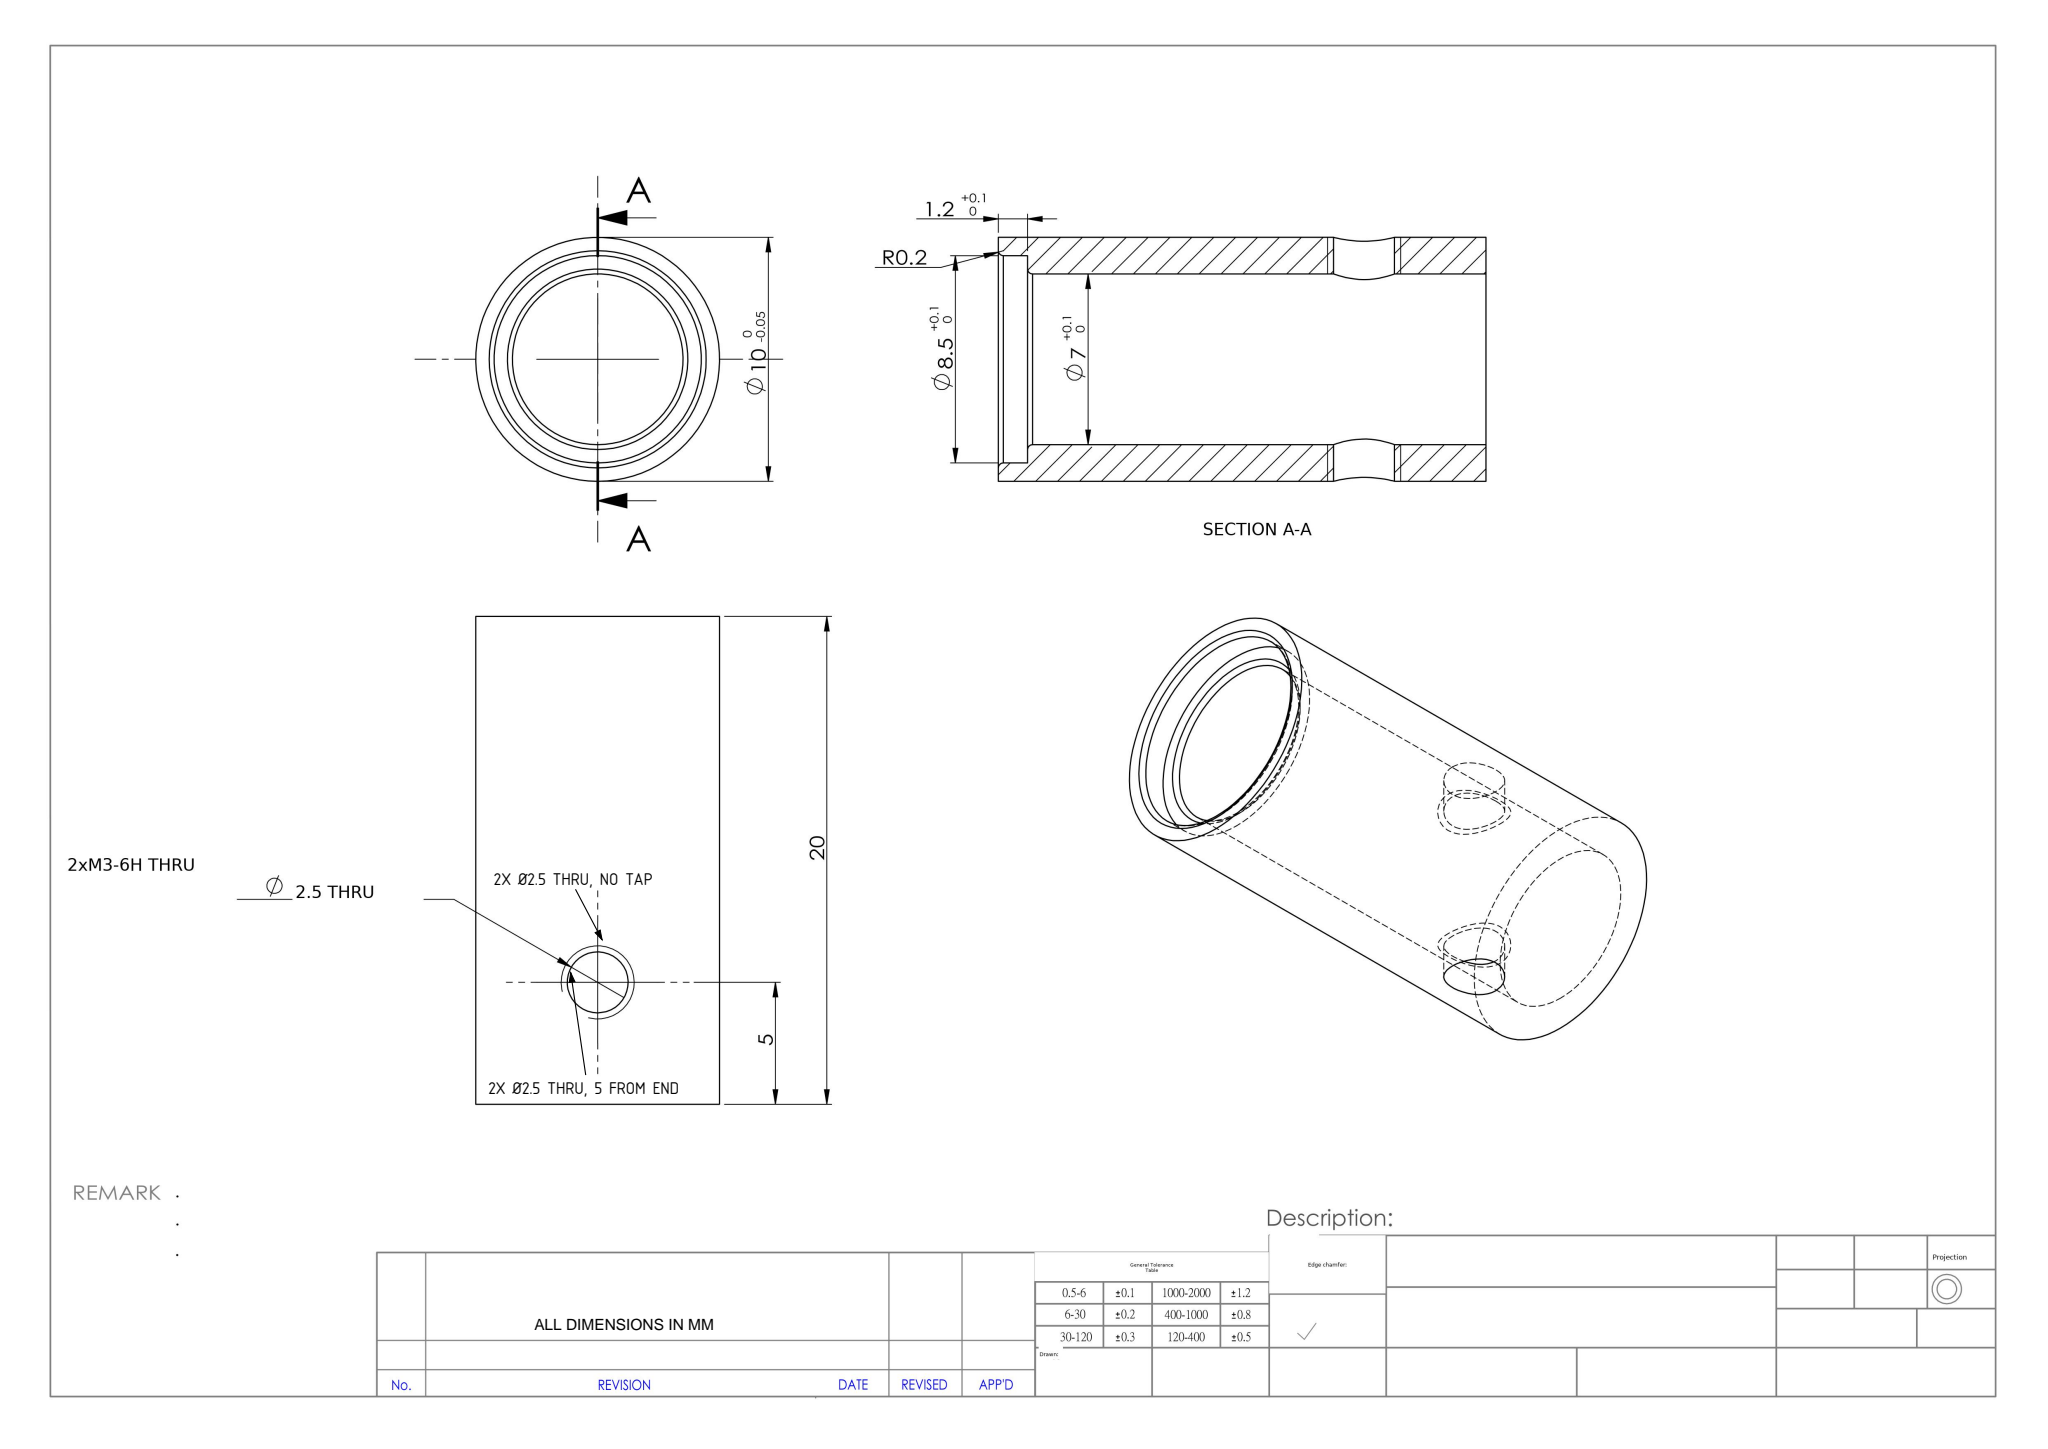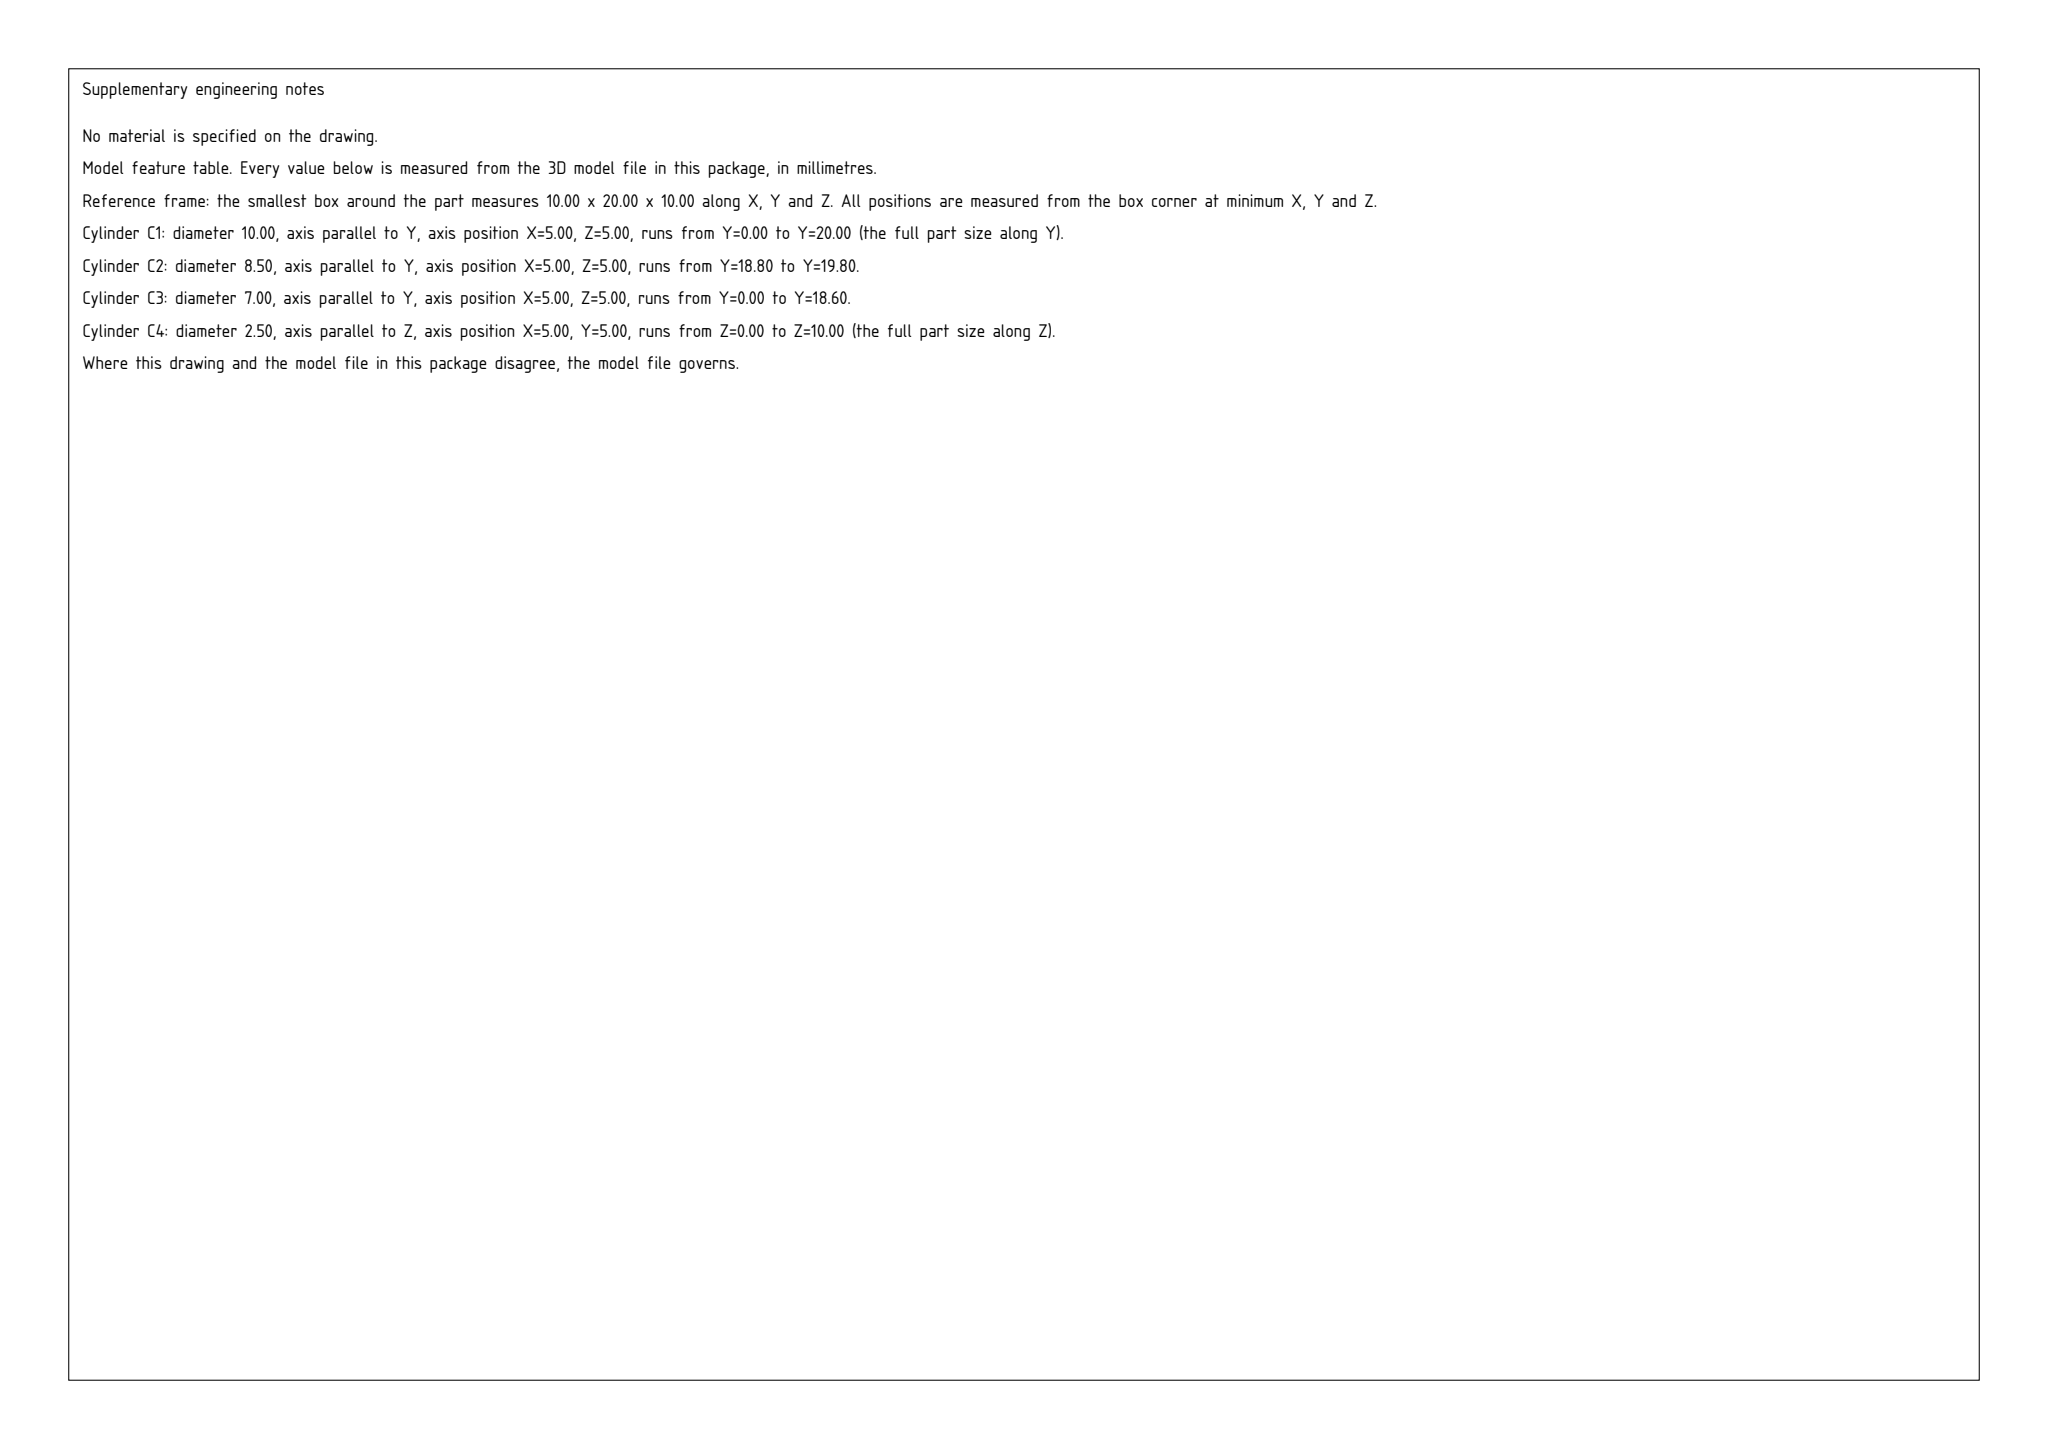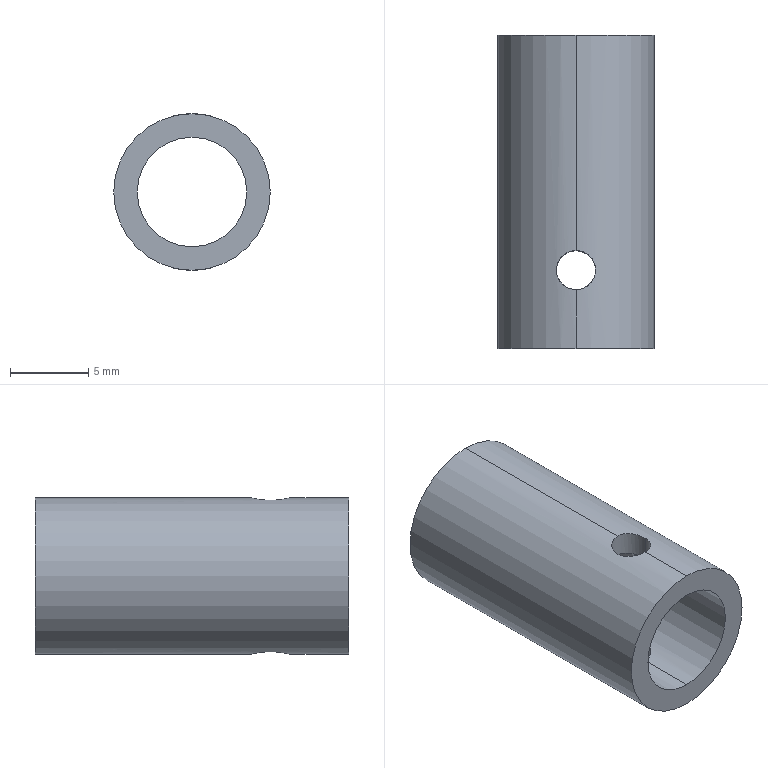Part | SolidWorks | mm | 1 solid | 17 faces | box 10 x 20 x 10 mm | volume 764 mm3 | cylinder 10 | torus 4 | plane 3 | commonest cylinder face diameters 2.5 x4 8.5 x2 10 x2 7 x2
Drawing notes:
2X Ø2.5 THRU WALL - NOT TAPPED (DELETE 2xM3-6H NOTE) | from the solid: Two Ø2.5 bores on z axis at x=5, y=5 (z 0-1.7 and 8.3-10); no thread/cone geometry in STEP
2X Ø2.5 THRU, ON C/L, 5 FROM BOTTOM END FACE | from the solid: Ø2.5 holes, axis z, located x=5.0 (Ø10 c/l), y=5.0 from y=0 end face; part length 20
build123d program:
from build123d import *

# Parameters (mm, degrees)
SKETCH7_R           = 5
BOSS_EXTRUDE3_DEPTH = 20
SKETCH8_R           = 3.5
CUT_EXTRUDE3_DEPTH  = 22.213
SKETCH9_R           = 4.25
CUT_EXTRUDE4_DEPTH  = 1.2
SKETCH14_W          = 1.25
SKETCH14_H          = 5
M3_TAPPED_HOLE2_D   = 2.5
FILLET1_R           = 0.2


with BuildPart() as part:
    # Sketch7 → Boss-Extrude3 (new body)
    with BuildSketch(Plane(origin=(0, 0, 0), x_dir=(1, 0, 0), z_dir=(0, 1, 0))):
        with Locations(Location((0, 0, 0), (0, 0, 270))):
            Circle(SKETCH7_R)
    extrude(amount=BOSS_EXTRUDE3_DEPTH)

    # Sketch8 → Cut-Extrude3 (cut, through all)
    with BuildSketch(Plane(origin=(0, 20, 0), x_dir=(1, 0, 0), z_dir=(0, 1, 0))):
        with Locations(Location((0, 0, 0), (0, 0, 270))):
            Circle(SKETCH8_R)
    extrude(amount=-CUT_EXTRUDE3_DEPTH, mode=Mode.SUBTRACT)

    # Sketch9 → Cut-Extrude4 (cut)
    with BuildSketch(Plane(origin=(0, 20, 0), x_dir=(1, 0, 0), z_dir=(0, 1, 0))):
        with Locations(Location((0, 0, 0), (0, 0, 270))):
            Circle(SKETCH9_R)
    extrude(amount=-CUT_EXTRUDE4_DEPTH, mode=Mode.SUBTRACT)

    # Sketch14 → M3 Tapped Hole1 (revolve, cut)
    with BuildSketch(Plane(origin=(0, 5, 0), x_dir=(0, 1, 0), z_dir=(1, 0, 0))):
        with Locations((0.625, 2.5)):
            Rectangle(SKETCH14_W, SKETCH14_H)
    revolve(axis=Axis((0, 5, -6.35), (0, 0, 1)), mode=Mode.SUBTRACT)

    # M3 Tapped Hole2 (through all)
    with Locations(Plane.XY):
        with Locations((0, 5)):
            Hole(M3_TAPPED_HOLE2_D / 2)

    # Fillet1
    fillet1_edges = [part.edges().sort_by_distance(p)[0] for p in [
        (0, 20, -4.25),
        (0, 18.8, -3.5),
    ]]
    fillet(fillet1_edges, radius=FILLET1_R)


solid = part.part
STEP:
#1=CARTESIAN_POINT('',(0.,18.8,-3.7));
#2=VERTEX_POINT('',#1);
#3=CARTESIAN_POINT('',(0.,18.8,3.7));
#4=VERTEX_POINT('',#3);
#5=CARTESIAN_POINT('',(0.,18.8,0.));
#6=DIRECTION('',(0.,-1.,0.));
#7=DIRECTION('',(0.,0.,1.));
#8=AXIS2_PLACEMENT_3D('',#5,#6,#7);
#9=CIRCLE('',#8,3.7);
#10=EDGE_CURVE('',#2,#4,#9,.T.);
#11=ORIENTED_EDGE('',*,*,#10,.F.);
#12=CARTESIAN_POINT('',(0.,18.6,-3.5));
#13=VERTEX_POINT('',#12);
#14=CARTESIAN_POINT('',(0.,18.6,-3.7));
#15=DIRECTION('',(1.,0.,0.));
#16=DIRECTION('',(0.,0.,-1.));
#17=AXIS2_PLACEMENT_3D('',#14,#15,#16);
#18=CIRCLE('',#17,0.2);
#19=EDGE_CURVE('',#2,#13,#18,.T.);
#20=ORIENTED_EDGE('',*,*,#19,.T.);
#21=CARTESIAN_POINT('',(0.,18.6,3.5));
#22=VERTEX_POINT('',#21);
#23=CARTESIAN_POINT('',(0.,18.6,0.));
#24=DIRECTION('',(0.,1.,0.));
#25=DIRECTION('',(0.,0.,1.));
#26=AXIS2_PLACEMENT_3D('',#23,#24,#25);
#27=CIRCLE('',#26,3.5);
#28=EDGE_CURVE('',#22,#13,#27,.T.);
#29=ORIENTED_EDGE('',*,*,#28,.F.);
#30=CARTESIAN_POINT('',(0.,18.6,3.7));
#31=DIRECTION('',(-1.,0.,0.));
#32=DIRECTION('',(0.,0.,1.));
#33=AXIS2_PLACEMENT_3D('',#30,#31,#32);
#34=CIRCLE('',#33,0.2);
#35=EDGE_CURVE('',#4,#22,#34,.T.);
#36=ORIENTED_EDGE('',*,*,#35,.F.);
#37=EDGE_LOOP('',(#11,#20,#29,#36));
#38=FACE_OUTER_BOUND('',#37,.T.);
#39=CARTESIAN_POINT('',(0.,18.6,0.));
#40=DIRECTION('',(0.,1.,0.));
#41=DIRECTION('',(0.,0.,1.));
#42=AXIS2_PLACEMENT_3D('',#39,#40,#41);
#43=TOROIDAL_SURFACE('',#42,3.7,0.2);
#44=ADVANCED_FACE('',(#38),#43,.T.);
#45=CARTESIAN_POINT('',(0.,20.,-4.45));
#46=VERTEX_POINT('',#45);
#47=CARTESIAN_POINT('',(0.,20.,4.45));
#48=VERTEX_POINT('',#47);
#49=CARTESIAN_POINT('',(0.,20.,0.));
#50=DIRECTION('',(0.,-1.,0.));
#51=DIRECTION('',(0.,0.,1.));
#52=AXIS2_PLACEMENT_3D('',#49,#50,#51);
#53=CIRCLE('',#52,4.45);
#54=EDGE_CURVE('',#46,#48,#53,.T.);
#55=ORIENTED_EDGE('',*,*,#54,.F.);
#56=CARTESIAN_POINT('',(0.,19.8,-4.25));
#57=VERTEX_POINT('',#56);
#58=CARTESIAN_POINT('',(0.,19.8,-4.45));
#59=DIRECTION('',(1.,0.,0.));
#60=DIRECTION('',(0.,0.,-1.));
#61=AXIS2_PLACEMENT_3D('',#58,#59,#60);
#62=CIRCLE('',#61,0.2);
#63=EDGE_CURVE('',#46,#57,#62,.T.);
#64=ORIENTED_EDGE('',*,*,#63,.T.);
#65=CARTESIAN_POINT('',(0.,19.8,4.25));
#66=VERTEX_POINT('',#65);
#67=CARTESIAN_POINT('',(0.,19.8,0.));
#68=DIRECTION('',(0.,1.,0.));
#69=DIRECTION('',(0.,0.,1.));
#70=AXIS2_PLACEMENT_3D('',#67,#68,#69);
#71=CIRCLE('',#70,4.25);
#72=EDGE_CURVE('',#66,#57,#71,.T.);
#73=ORIENTED_EDGE('',*,*,#72,.F.);
#74=CARTESIAN_POINT('',(0.,19.8,4.45));
#75=DIRECTION('',(-1.,0.,0.));
#76=DIRECTION('',(0.,0.,1.));
#77=AXIS2_PLACEMENT_3D('',#74,#75,#76);
#78=CIRCLE('',#77,0.2);
#79=EDGE_CURVE('',#48,#66,#78,.T.);
#80=ORIENTED_EDGE('',*,*,#79,.F.);
#81=EDGE_LOOP('',(#55,#64,#73,#80));
#82=FACE_OUTER_BOUND('',#81,.T.);
#83=CARTESIAN_POINT('',(0.,19.8,0.));
#84=DIRECTION('',(0.,1.,0.));
#85=DIRECTION('',(0.,0.,1.));
#86=AXIS2_PLACEMENT_3D('',#83,#84,#85);
#87=TOROIDAL_SURFACE('',#86,4.45,0.2);
#88=ADVANCED_FACE('',(#82),#87,.T.);
#89=CARTESIAN_POINT('',(-1.25,5.,-4.841));
#90=VERTEX_POINT('',#89);
#91=CARTESIAN_POINT('',(0.,3.75,-5.));
#92=VERTEX_POINT('',#91);
#93=CARTESIAN_POINT('',(-1.25,5.,-4.841));
#94=CARTESIAN_POINT('',(-1.25,4.918,-4.841));
#95=CARTESIAN_POINT('',(-1.242,4.835,-4.843));
#96=CARTESIAN_POINT('',(-1.21,4.674,-4.852));
#97=CARTESIAN_POINT('',(-1.186,4.596,-4.857));
#98=CARTESIAN_POINT('',(-1.091,4.369,-4.88));
#99=CARTESIAN_POINT('',(-0.9993,4.231,-4.901));
#100=CARTESIAN_POINT('',(-0.8256,4.058,-4.932));
#101=CARTESIAN_POINT('',(-0.7628,4.006,-4.942));
#102=CARTESIAN_POINT('',(-0.6277,3.916,-4.961));
#103=CARTESIAN_POINT('',(-0.5545,3.877,-4.97));
#104=CARTESIAN_POINT('',(-0.3282,3.783,-4.992));
#105=CARTESIAN_POINT('',(-0.1635,3.75,-5.));
#106=CARTESIAN_POINT('',(0.,3.75,-5.));
#107=B_SPLINE_CURVE_WITH_KNOTS('',3,(#93,#94,#95,#96,#97,#98,#99,#100,#101,#102,#103,#104,#105,#106),.UNSPECIFIED.,.F.,.F.,(4,2,2,2,2,2,4),(0.001962,0.002208,0.002453,0.002943,0.003188,0.003433,0.003924),.UNSPECIFIED.);
#108=EDGE_CURVE('',#90,#92,#107,.T.);
#109=ORIENTED_EDGE('',*,*,#108,.F.);
#110=CARTESIAN_POINT('',(-1.25,5.,-3.269));
#111=VERTEX_POINT('',#110);
#112=CARTESIAN_POINT('',(-1.25,5.,0.));
#113=DIRECTION('',(0.,0.,1.));
#114=VECTOR('',#113,1000.);
#115=LINE('',#112,#114);
#116=EDGE_CURVE('',#90,#111,#115,.T.);
#117=ORIENTED_EDGE('',*,*,#116,.T.);
#118=CARTESIAN_POINT('',(-0.,3.75,-3.5));
#119=VERTEX_POINT('',#118);
#120=CARTESIAN_POINT('',(-0.,3.75,-3.5));
#121=CARTESIAN_POINT('',(-0.08231,3.75,-3.5));
#122=CARTESIAN_POINT('',(-0.1659,3.758,-3.497));
#123=CARTESIAN_POINT('',(-0.3268,3.791,-3.486));
#124=CARTESIAN_POINT('',(-0.405,3.815,-3.477));
#125=CARTESIAN_POINT('',(-0.6334,3.91,-3.446));
#126=CARTESIAN_POINT('',(-0.7701,4.002,-3.416));
#127=CARTESIAN_POINT('',(-0.9421,4.174,-3.371));
#128=CARTESIAN_POINT('',(-0.9934,4.237,-3.356));
#129=CARTESIAN_POINT('',(-1.084,4.372,-3.328));
#130=CARTESIAN_POINT('',(-1.123,4.445,-3.315));
#131=CARTESIAN_POINT('',(-1.217,4.67,-3.282));
#132=CARTESIAN_POINT('',(-1.25,4.836,-3.269));
#133=CARTESIAN_POINT('',(-1.25,5.,-3.269));
#134=B_SPLINE_CURVE_WITH_KNOTS('',3,(#120,#121,#122,#123,#124,#125,#126,#127,#128,#129,#130,#131,#132,#133),.UNSPECIFIED.,.F.,.F.,(4,2,2,2,2,2,4),(0.001971,0.002217,0.002463,0.002956,0.003202,0.003448,0.003941),.UNSPECIFIED.);
#135=EDGE_CURVE('',#119,#111,#134,.T.);
#136=ORIENTED_EDGE('',*,*,#135,.F.);
#137=CARTESIAN_POINT('',(1.25,5.,-3.269));
#138=VERTEX_POINT('',#137);
#139=CARTESIAN_POINT('',(1.25,5.,-3.269));
#140=CARTESIAN_POINT('',(1.25,4.833,-3.269));
#141=CARTESIAN_POINT('',(1.217,4.67,-3.282));
#142=CARTESIAN_POINT('',(1.091,4.368,-3.326));
#143=CARTESIAN_POINT('',(0.9979,4.23,-3.357));
#144=CARTESIAN_POINT('',(0.7692,4.002,-3.416));
#145=CARTESIAN_POINT('',(0.6308,3.909,-3.446));
#146=CARTESIAN_POINT('',(0.3302,3.783,-3.488));
#147=CARTESIAN_POINT('',(0.1647,3.75,-3.5));
#148=CARTESIAN_POINT('',(-0.,3.75,-3.5));
#149=B_SPLINE_CURVE_WITH_KNOTS('',3,(#139,#140,#141,#142,#143,#144,#145,#146,#147,#148),.UNSPECIFIED.,.F.,.F.,(4,2,2,2,4),(0.,0.0004927,0.0009855,0.001478,0.001971),.UNSPECIFIED.);
#150=EDGE_CURVE('',#138,#119,#149,.T.);
#151=ORIENTED_EDGE('',*,*,#150,.F.);
#152=CARTESIAN_POINT('',(1.25,5.,-4.841));
#153=VERTEX_POINT('',#152);
#154=CARTESIAN_POINT('',(1.25,5.,0.));
#155=DIRECTION('',(0.,0.,1.));
#156=VECTOR('',#155,1000.);
#157=LINE('',#154,#156);
#158=EDGE_CURVE('',#153,#138,#157,.T.);
#159=ORIENTED_EDGE('',*,*,#158,.F.);
#160=CARTESIAN_POINT('',(0.,3.75,-5.));
#161=CARTESIAN_POINT('',(0.1635,3.75,-5.));
#162=CARTESIAN_POINT('',(0.3287,3.783,-4.991));
#163=CARTESIAN_POINT('',(0.6298,3.908,-4.962));
#164=CARTESIAN_POINT('',(0.7684,4.001,-4.942));
#165=CARTESIAN_POINT('',(0.999,4.231,-4.901));
#166=CARTESIAN_POINT('',(1.091,4.368,-4.88));
#167=CARTESIAN_POINT('',(1.217,4.672,-4.85));
#168=CARTESIAN_POINT('',(1.25,4.835,-4.841));
#169=CARTESIAN_POINT('',(1.25,5.,-4.841));
#170=B_SPLINE_CURVE_WITH_KNOTS('',3,(#160,#161,#162,#163,#164,#165,#166,#167,#168,#169),.UNSPECIFIED.,.F.,.F.,(4,2,2,2,4),(0.003924,0.004414,0.004905,0.005395,0.005885),.UNSPECIFIED.);
#171=EDGE_CURVE('',#92,#153,#170,.T.);
#172=ORIENTED_EDGE('',*,*,#171,.F.);
#173=EDGE_LOOP('',(#109,#117,#136,#151,#159,#172));
#174=FACE_OUTER_BOUND('',#173,.T.);
#175=CARTESIAN_POINT('',(0.,5.,0.));
#176=DIRECTION('',(0.,0.,1.));
#177=DIRECTION('',(1.,0.,0.));
#178=AXIS2_PLACEMENT_3D('',#175,#176,#177);
#179=CYLINDRICAL_SURFACE('',#178,1.25);
#180=ADVANCED_FACE('',(#174),#179,.F.);
#181=CARTESIAN_POINT('',(1.25,5.,4.841));
#182=VERTEX_POINT('',#181);
#183=CARTESIAN_POINT('',(0.,3.75,5.));
#184=VERTEX_POINT('',#183);
#185=CARTESIAN_POINT('',(1.25,5.,4.841));
#186=CARTESIAN_POINT('',(1.25,4.918,4.841));
#187=CARTESIAN_POINT('',(1.242,4.836,4.843));
#188=CARTESIAN_POINT('',(1.21,4.676,4.851));
#189=CARTESIAN_POINT('',(1.186,4.596,4.857));
#190=CARTESIAN_POINT('',(1.092,4.37,4.88));
#191=CARTESIAN_POINT('',(0.9989,4.231,4.901));
#192=CARTESIAN_POINT('',(0.7696,4.002,4.942));
#193=CARTESIAN_POINT('',(0.6309,3.909,4.962));
#194=CARTESIAN_POINT('',(0.3301,3.783,4.991));
#195=CARTESIAN_POINT('',(0.1658,3.75,5.));
#196=CARTESIAN_POINT('',(0.,3.75,5.));
#197=B_SPLINE_CURVE_WITH_KNOTS('',3,(#185,#186,#187,#188,#189,#190,#191,#192,#193,#194,#195,#196),.UNSPECIFIED.,.F.,.F.,(4,2,2,2,2,4),(0.005885,0.006131,0.006376,0.006866,0.007356,0.007846),.UNSPECIFIED.);
#198=EDGE_CURVE('',#182,#184,#197,.T.);
#199=ORIENTED_EDGE('',*,*,#198,.F.);
#200=CARTESIAN_POINT('',(1.25,5.,3.269));
#201=VERTEX_POINT('',#200);
#202=CARTESIAN_POINT('',(1.25,5.,0.));
#203=DIRECTION('',(0.,0.,-1.));
#204=VECTOR('',#203,1000.);
#205=LINE('',#202,#204);
#206=EDGE_CURVE('',#182,#201,#205,.T.);
#207=ORIENTED_EDGE('',*,*,#206,.T.);
#208=CARTESIAN_POINT('',(0.,3.75,3.5));
#209=VERTEX_POINT('',#208);
#210=CARTESIAN_POINT('',(0.,3.75,3.5));
#211=CARTESIAN_POINT('',(0.1667,3.75,3.5));
#212=CARTESIAN_POINT('',(0.3302,3.783,3.488));
#213=CARTESIAN_POINT('',(0.6325,3.909,3.446));
#214=CARTESIAN_POINT('',(0.7703,4.002,3.416));
#215=CARTESIAN_POINT('',(0.9988,4.231,3.357));
#216=CARTESIAN_POINT('',(1.092,4.37,3.326));
#217=CARTESIAN_POINT('',(1.217,4.67,3.282));
#218=CARTESIAN_POINT('',(1.25,4.835,3.269));
#219=CARTESIAN_POINT('',(1.25,5.,3.269));
#220=B_SPLINE_CURVE_WITH_KNOTS('',3,(#210,#211,#212,#213,#214,#215,#216,#217,#218,#219),.UNSPECIFIED.,.F.,.F.,(4,2,2,2,4),(0.,0.0004928,0.0009856,0.001478,0.001971),.UNSPECIFIED.);
#221=EDGE_CURVE('',#209,#201,#220,.T.);
#222=ORIENTED_EDGE('',*,*,#221,.F.);
#223=CARTESIAN_POINT('',(-1.25,5.,3.269));
#224=VERTEX_POINT('',#223);
#225=CARTESIAN_POINT('',(-1.25,5.,3.269));
#226=CARTESIAN_POINT('',(-1.25,4.835,3.269));
#227=CARTESIAN_POINT('',(-1.217,4.67,3.282));
#228=CARTESIAN_POINT('',(-1.091,4.369,3.326));
#229=CARTESIAN_POINT('',(-0.9986,4.231,3.357));
#230=CARTESIAN_POINT('',(-0.7693,4.002,3.416));
#231=CARTESIAN_POINT('',(-0.6323,3.909,3.446));
#232=CARTESIAN_POINT('',(-0.3293,3.783,3.488));
#233=CARTESIAN_POINT('',(-0.1667,3.75,3.5));
#234=CARTESIAN_POINT('',(0.,3.75,3.5));
#235=B_SPLINE_CURVE_WITH_KNOTS('',3,(#225,#226,#227,#228,#229,#230,#231,#232,#233,#234),.UNSPECIFIED.,.F.,.F.,(4,2,2,2,4),(0.005911,0.006403,0.006896,0.007388,0.007881),.UNSPECIFIED.);
#236=EDGE_CURVE('',#224,#209,#235,.T.);
#237=ORIENTED_EDGE('',*,*,#236,.F.);
#238=CARTESIAN_POINT('',(-1.25,5.,4.841));
#239=VERTEX_POINT('',#238);
#240=CARTESIAN_POINT('',(-1.25,5.,0.));
#241=DIRECTION('',(0.,0.,-1.));
#242=VECTOR('',#241,1000.);
#243=LINE('',#240,#242);
#244=EDGE_CURVE('',#239,#224,#243,.T.);
#245=ORIENTED_EDGE('',*,*,#244,.F.);
#246=CARTESIAN_POINT('',(0.,3.75,5.));
#247=CARTESIAN_POINT('',(-0.1659,3.75,5.));
#248=CARTESIAN_POINT('',(-0.3287,3.783,4.991));
#249=CARTESIAN_POINT('',(-0.6313,3.909,4.962));
#250=CARTESIAN_POINT('',(-0.7695,4.002,4.942));
#251=CARTESIAN_POINT('',(-0.9991,4.231,4.901));
#252=CARTESIAN_POINT('',(-1.092,4.37,4.88));
#253=CARTESIAN_POINT('',(-1.217,4.671,4.85));
#254=CARTESIAN_POINT('',(-1.25,4.836,4.841));
#255=CARTESIAN_POINT('',(-1.25,5.,4.841));
#256=B_SPLINE_CURVE_WITH_KNOTS('',3,(#246,#247,#248,#249,#250,#251,#252,#253,#254,#255),.UNSPECIFIED.,.F.,.F.,(4,2,2,2,4),(0.,0.0004906,0.0009812,0.001472,0.001962),.UNSPECIFIED.);
#257=EDGE_CURVE('',#184,#239,#256,.T.);
#258=ORIENTED_EDGE('',*,*,#257,.F.);
#259=EDGE_LOOP('',(#199,#207,#222,#237,#245,#258));
#260=FACE_OUTER_BOUND('',#259,.T.);
#261=CARTESIAN_POINT('',(0.,5.,0.));
#262=DIRECTION('',(0.,0.,-1.));
#263=DIRECTION('',(-1.,0.,0.));
#264=AXIS2_PLACEMENT_3D('',#261,#262,#263);
#265=CYLINDRICAL_SURFACE('',#264,1.25);
#266=ADVANCED_FACE('',(#260),#265,.F.);
#267=CARTESIAN_POINT('',(0.,18.8,-4.25));
#268=VERTEX_POINT('',#267);
#269=CARTESIAN_POINT('',(0.,18.8,4.25));
#270=VERTEX_POINT('',#269);
#271=CARTESIAN_POINT('',(0.,18.8,0.));
#272=DIRECTION('',(0.,1.,0.));
#273=DIRECTION('',(0.,0.,1.));
#274=AXIS2_PLACEMENT_3D('',#271,#272,#273);
#275=CIRCLE('',#274,4.25);
#276=EDGE_CURVE('',#268,#270,#275,.T.);
#277=ORIENTED_EDGE('',*,*,#276,.F.);
#278=CARTESIAN_POINT('',(0.,18.8,-4.25));
#279=DIRECTION('',(0.,1.,0.));
#280=VECTOR('',#279,1000.);
#281=LINE('',#278,#280);
#282=EDGE_CURVE('',#268,#57,#281,.T.);
#283=ORIENTED_EDGE('',*,*,#282,.T.);
#284=CARTESIAN_POINT('',(0.,19.8,0.));
#285=DIRECTION('',(0.,1.,0.));
#286=DIRECTION('',(0.,0.,1.));
#287=AXIS2_PLACEMENT_3D('',#284,#285,#286);
#288=CIRCLE('',#287,4.25);
#289=EDGE_CURVE('',#57,#66,#288,.T.);
#290=ORIENTED_EDGE('',*,*,#289,.T.);
#291=CARTESIAN_POINT('',(0.,18.8,4.25));
#292=DIRECTION('',(0.,1.,0.));
#293=VECTOR('',#292,1000.);
#294=LINE('',#291,#293);
#295=EDGE_CURVE('',#270,#66,#294,.T.);
#296=ORIENTED_EDGE('',*,*,#295,.F.);
#297=EDGE_LOOP('',(#277,#283,#290,#296));
#298=FACE_OUTER_BOUND('',#297,.T.);
#299=CARTESIAN_POINT('',(0.,18.8,0.));
#300=DIRECTION('',(0.,1.,0.));
#301=DIRECTION('',(0.,0.,1.));
#302=AXIS2_PLACEMENT_3D('',#299,#300,#301);
#303=CYLINDRICAL_SURFACE('',#302,4.25);
#304=ADVANCED_FACE('',(#298),#303,.F.);
#305=CARTESIAN_POINT('',(0.,20.,5.));
#306=VERTEX_POINT('',#305);
#307=CARTESIAN_POINT('',(0.,20.,-5.));
#308=VERTEX_POINT('',#307);
#309=CARTESIAN_POINT('',(0.,20.,0.));
#310=DIRECTION('',(0.,1.,0.));
#311=DIRECTION('',(0.,0.,1.));
#312=AXIS2_PLACEMENT_3D('',#309,#310,#311);
#313=CIRCLE('',#312,5.);
#314=EDGE_CURVE('',#306,#308,#313,.T.);
#315=ORIENTED_EDGE('',*,*,#314,.F.);
#316=CARTESIAN_POINT('',(0.,6.25,5.));
#317=VERTEX_POINT('',#316);
#318=CARTESIAN_POINT('',(0.,20.,5.));
#319=DIRECTION('',(0.,-1.,0.));
#320=VECTOR('',#319,1000.);
#321=LINE('',#318,#320);
#322=EDGE_CURVE('',#306,#317,#321,.T.);
#323=ORIENTED_EDGE('',*,*,#322,.T.);
#324=CARTESIAN_POINT('',(0.,6.25,5.));
#325=CARTESIAN_POINT('',(0.1635,6.25,5.));
#326=CARTESIAN_POINT('',(0.3287,6.217,4.991));
#327=CARTESIAN_POINT('',(0.6298,6.092,4.962));
#328=CARTESIAN_POINT('',(0.7684,5.999,4.942));
#329=CARTESIAN_POINT('',(0.999,5.769,4.901));
#330=CARTESIAN_POINT('',(1.091,5.632,4.88));
#331=CARTESIAN_POINT('',(1.217,5.328,4.85));
#332=CARTESIAN_POINT('',(1.25,5.165,4.841));
#333=CARTESIAN_POINT('',(1.25,5.,4.841));
#334=B_SPLINE_CURVE_WITH_KNOTS('',3,(#324,#325,#326,#327,#328,#329,#330,#331,#332,#333),.UNSPECIFIED.,.F.,.F.,(4,2,2,2,4),(0.003924,0.004414,0.004905,0.005395,0.005885),.UNSPECIFIED.);
#335=EDGE_CURVE('',#317,#182,#334,.T.);
#336=ORIENTED_EDGE('',*,*,#335,.T.);
#337=ORIENTED_EDGE('',*,*,#198,.T.);
#338=CARTESIAN_POINT('',(0.,0.,5.));
#339=VERTEX_POINT('',#338);
#340=CARTESIAN_POINT('',(0.,20.,5.));
#341=DIRECTION('',(0.,-1.,0.));
#342=VECTOR('',#341,1000.);
#343=LINE('',#340,#342);
#344=EDGE_CURVE('',#184,#339,#343,.T.);
#345=ORIENTED_EDGE('',*,*,#344,.T.);
#346=CARTESIAN_POINT('',(0.,0.,-5.));
#347=VERTEX_POINT('',#346);
#348=CARTESIAN_POINT('',(0.,0.,0.));
#349=DIRECTION('',(0.,1.,0.));
#350=DIRECTION('',(0.,0.,1.));
#351=AXIS2_PLACEMENT_3D('',#348,#349,#350);
#352=CIRCLE('',#351,5.);
#353=EDGE_CURVE('',#339,#347,#352,.T.);
#354=ORIENTED_EDGE('',*,*,#353,.T.);
#355=CARTESIAN_POINT('',(0.,20.,-5.));
#356=DIRECTION('',(0.,-1.,0.));
#357=VECTOR('',#356,1000.);
#358=LINE('',#355,#357);
#359=EDGE_CURVE('',#92,#347,#358,.T.);
#360=ORIENTED_EDGE('',*,*,#359,.F.);
#361=ORIENTED_EDGE('',*,*,#171,.T.);
#362=CARTESIAN_POINT('',(-0.,6.25,-5.));
#363=VERTEX_POINT('',#362);
#364=CARTESIAN_POINT('',(1.25,5.,-4.841));
#365=CARTESIAN_POINT('',(1.25,5.082,-4.841));
#366=CARTESIAN_POINT('',(1.242,5.164,-4.843));
#367=CARTESIAN_POINT('',(1.21,5.324,-4.851));
#368=CARTESIAN_POINT('',(1.186,5.404,-4.857));
#369=CARTESIAN_POINT('',(1.092,5.63,-4.88));
#370=CARTESIAN_POINT('',(0.9989,5.769,-4.901));
#371=CARTESIAN_POINT('',(0.7696,5.998,-4.942));
#372=CARTESIAN_POINT('',(0.6309,6.091,-4.962));
#373=CARTESIAN_POINT('',(0.3301,6.217,-4.991));
#374=CARTESIAN_POINT('',(0.1658,6.25,-5.));
#375=CARTESIAN_POINT('',(-0.,6.25,-5.));
#376=B_SPLINE_CURVE_WITH_KNOTS('',3,(#364,#365,#366,#367,#368,#369,#370,#371,#372,#373,#374,#375),.UNSPECIFIED.,.F.,.F.,(4,2,2,2,2,4),(0.005885,0.006131,0.006376,0.006866,0.007356,0.007846),.UNSPECIFIED.);
#377=EDGE_CURVE('',#153,#363,#376,.T.);
#378=ORIENTED_EDGE('',*,*,#377,.T.);
#379=CARTESIAN_POINT('',(0.,20.,-5.));
#380=DIRECTION('',(0.,-1.,0.));
#381=VECTOR('',#380,1000.);
#382=LINE('',#379,#381);
#383=EDGE_CURVE('',#308,#363,#382,.T.);
#384=ORIENTED_EDGE('',*,*,#383,.F.);
#385=EDGE_LOOP('',(#315,#323,#336,#337,#345,#354,#360,#361,#378,#384));
#386=FACE_OUTER_BOUND('',#385,.T.);
#387=CARTESIAN_POINT('',(0.,20.,0.));
#388=DIRECTION('',(0.,-1.,0.));
#389=DIRECTION('',(0.,0.,-1.));
#390=AXIS2_PLACEMENT_3D('',#387,#388,#389);
#391=CYLINDRICAL_SURFACE('',#390,5.);
#392=ADVANCED_FACE('',(#386),#391,.T.);
#393=CARTESIAN_POINT('',(0.,0.,-3.5));
#394=VERTEX_POINT('',#393);
#395=CARTESIAN_POINT('',(0.,0.,3.5));
#396=VERTEX_POINT('',#395);
#397=CARTESIAN_POINT('',(0.,0.,0.));
#398=DIRECTION('',(0.,1.,0.));
#399=DIRECTION('',(0.,0.,1.));
#400=AXIS2_PLACEMENT_3D('',#397,#398,#399);
#401=CIRCLE('',#400,3.5);
#402=EDGE_CURVE('',#394,#396,#401,.T.);
#403=ORIENTED_EDGE('',*,*,#402,.F.);
#404=CARTESIAN_POINT('',(0.,0.,-3.5));
#405=DIRECTION('',(0.,1.,0.));
#406=VECTOR('',#405,1000.);
#407=LINE('',#404,#406);
#408=EDGE_CURVE('',#394,#119,#407,.T.);
#409=ORIENTED_EDGE('',*,*,#408,.T.);
#410=ORIENTED_EDGE('',*,*,#135,.T.);
#411=CARTESIAN_POINT('',(-0.,6.25,-3.5));
#412=VERTEX_POINT('',#411);
#413=CARTESIAN_POINT('',(-1.25,5.,-3.269));
#414=CARTESIAN_POINT('',(-1.25,5.164,-3.269));
#415=CARTESIAN_POINT('',(-1.217,5.33,-3.282));
#416=CARTESIAN_POINT('',(-1.091,5.631,-3.326));
#417=CARTESIAN_POINT('',(-0.9994,5.768,-3.356));
#418=CARTESIAN_POINT('',(-0.7684,5.999,-3.417));
#419=CARTESIAN_POINT('',(-0.6321,6.091,-3.446));
#420=CARTESIAN_POINT('',(-0.4047,6.186,-3.477));
#421=CARTESIAN_POINT('',(-0.3266,6.209,-3.486));
#422=CARTESIAN_POINT('',(-0.1659,6.242,-3.497));
#423=CARTESIAN_POINT('',(-0.08235,6.25,-3.5));
#424=CARTESIAN_POINT('',(-0.,6.25,-3.5));
#425=B_SPLINE_CURVE_WITH_KNOTS('',3,(#413,#414,#415,#416,#417,#418,#419,#420,#421,#422,#423,#424),.UNSPECIFIED.,.F.,.F.,(4,2,2,2,2,4),(0.003941,0.004433,0.004926,0.005418,0.005664,0.00591),.UNSPECIFIED.);
#426=EDGE_CURVE('',#111,#412,#425,.T.);
#427=ORIENTED_EDGE('',*,*,#426,.T.);
#428=CARTESIAN_POINT('',(0.,0.,-3.5));
#429=DIRECTION('',(0.,1.,0.));
#430=VECTOR('',#429,1000.);
#431=LINE('',#428,#430);
#432=EDGE_CURVE('',#412,#13,#431,.T.);
#433=ORIENTED_EDGE('',*,*,#432,.T.);
#434=CARTESIAN_POINT('',(0.,18.6,0.));
#435=DIRECTION('',(0.,1.,0.));
#436=DIRECTION('',(0.,0.,1.));
#437=AXIS2_PLACEMENT_3D('',#434,#435,#436);
#438=CIRCLE('',#437,3.5);
#439=EDGE_CURVE('',#13,#22,#438,.T.);
#440=ORIENTED_EDGE('',*,*,#439,.T.);
#441=CARTESIAN_POINT('',(0.,6.25,3.5));
#442=VERTEX_POINT('',#441);
#443=CARTESIAN_POINT('',(0.,0.,3.5));
#444=DIRECTION('',(0.,1.,0.));
#445=VECTOR('',#444,1000.);
#446=LINE('',#443,#445);
#447=EDGE_CURVE('',#442,#22,#446,.T.);
#448=ORIENTED_EDGE('',*,*,#447,.F.);
#449=CARTESIAN_POINT('',(0.,6.25,3.5));
#450=CARTESIAN_POINT('',(-0.1641,6.25,3.5));
#451=CARTESIAN_POINT('',(-0.3297,6.217,3.488));
#452=CARTESIAN_POINT('',(-0.6316,6.091,3.446));
#453=CARTESIAN_POINT('',(-0.7687,5.999,3.417));
#454=CARTESIAN_POINT('',(-0.9996,5.768,3.356));
#455=CARTESIAN_POINT('',(-1.091,5.632,3.326));
#456=CARTESIAN_POINT('',(-1.186,5.405,3.293));
#457=CARTESIAN_POINT('',(-1.209,5.327,3.284));
#458=CARTESIAN_POINT('',(-1.242,5.166,3.272));
#459=CARTESIAN_POINT('',(-1.25,5.082,3.269));
#460=CARTESIAN_POINT('',(-1.25,5.,3.269));
#461=B_SPLINE_CURVE_WITH_KNOTS('',3,(#449,#450,#451,#452,#453,#454,#455,#456,#457,#458,#459,#460),.UNSPECIFIED.,.F.,.F.,(4,2,2,2,2,4),(0.003941,0.004433,0.004926,0.005418,0.005664,0.005911),.UNSPECIFIED.);
#462=EDGE_CURVE('',#442,#224,#461,.T.);
#463=ORIENTED_EDGE('',*,*,#462,.T.);
#464=ORIENTED_EDGE('',*,*,#236,.T.);
#465=CARTESIAN_POINT('',(0.,0.,3.5));
#466=DIRECTION('',(0.,1.,0.));
#467=VECTOR('',#466,1000.);
#468=LINE('',#465,#467);
#469=EDGE_CURVE('',#396,#209,#468,.T.);
#470=ORIENTED_EDGE('',*,*,#469,.F.);
#471=EDGE_LOOP('',(#403,#409,#410,#427,#433,#440,#448,#463,#464,#470));
#472=FACE_OUTER_BOUND('',#471,.T.);
#473=CARTESIAN_POINT('',(0.,0.,0.));
#474=DIRECTION('',(0.,1.,0.));
#475=DIRECTION('',(0.,0.,1.));
#476=AXIS2_PLACEMENT_3D('',#473,#474,#475);
#477=CYLINDRICAL_SURFACE('',#476,3.5);
#478=ADVANCED_FACE('',(#472),#477,.F.);
#479=ORIENTED_EDGE('',*,*,#408,.F.);
#480=CARTESIAN_POINT('',(0.,0.,0.));
#481=DIRECTION('',(0.,1.,0.));
#482=DIRECTION('',(0.,0.,1.));
#483=AXIS2_PLACEMENT_3D('',#480,#481,#482);
#484=CIRCLE('',#483,3.5);
#485=EDGE_CURVE('',#396,#394,#484,.T.);
#486=ORIENTED_EDGE('',*,*,#485,.F.);
#487=ORIENTED_EDGE('',*,*,#469,.T.);
#488=ORIENTED_EDGE('',*,*,#221,.T.);
#489=CARTESIAN_POINT('',(1.25,5.,3.269));
#490=CARTESIAN_POINT('',(1.25,5.082,3.269));
#491=CARTESIAN_POINT('',(1.242,5.166,3.272));
#492=CARTESIAN_POINT('',(1.209,5.327,3.284));
#493=CARTESIAN_POINT('',(1.185,5.405,3.293));
#494=CARTESIAN_POINT('',(1.09,5.633,3.327));
#495=CARTESIAN_POINT('',(0.9982,5.77,3.357));
#496=CARTESIAN_POINT('',(0.8259,5.942,3.402));
#497=CARTESIAN_POINT('',(0.7635,5.993,3.416));
#498=CARTESIAN_POINT('',(0.6284,6.084,3.444));
#499=CARTESIAN_POINT('',(0.5554,6.123,3.456));
#500=CARTESIAN_POINT('',(0.3298,6.217,3.488));
#501=CARTESIAN_POINT('',(0.1641,6.25,3.5));
#502=CARTESIAN_POINT('',(0.,6.25,3.5));
#503=B_SPLINE_CURVE_WITH_KNOTS('',3,(#489,#490,#491,#492,#493,#494,#495,#496,#497,#498,#499,#500,#501,#502),.UNSPECIFIED.,.F.,.F.,(4,2,2,2,2,2,4),(0.001971,0.002217,0.002464,0.002956,0.003202,0.003448,0.003941),.UNSPECIFIED.);
#504=EDGE_CURVE('',#201,#442,#503,.T.);
#505=ORIENTED_EDGE('',*,*,#504,.T.);
#506=ORIENTED_EDGE('',*,*,#447,.T.);
#507=ORIENTED_EDGE('',*,*,#28,.T.);
#508=ORIENTED_EDGE('',*,*,#432,.F.);
#509=CARTESIAN_POINT('',(-0.,6.25,-3.5));
#510=CARTESIAN_POINT('',(0.1648,6.25,-3.5));
#511=CARTESIAN_POINT('',(0.3302,6.217,-3.488));
#512=CARTESIAN_POINT('',(0.6314,6.091,-3.446));
#513=CARTESIAN_POINT('',(0.7696,5.998,-3.416));
#514=CARTESIAN_POINT('',(0.9987,5.769,-3.357));
#515=CARTESIAN_POINT('',(1.091,5.632,-3.326));
#516=CARTESIAN_POINT('',(1.217,5.329,-3.282));
#517=CARTESIAN_POINT('',(1.25,5.167,-3.269));
#518=CARTESIAN_POINT('',(1.25,5.,-3.269));
#519=B_SPLINE_CURVE_WITH_KNOTS('',3,(#509,#510,#511,#512,#513,#514,#515,#516,#517,#518),.UNSPECIFIED.,.F.,.F.,(4,2,2,2,4),(0.00591,0.006403,0.006895,0.007388,0.007881),.UNSPECIFIED.);
#520=EDGE_CURVE('',#412,#138,#519,.T.);
#521=ORIENTED_EDGE('',*,*,#520,.T.);
#522=ORIENTED_EDGE('',*,*,#150,.T.);
#523=EDGE_LOOP('',(#479,#486,#487,#488,#505,#506,#507,#508,#521,#522));
#524=FACE_OUTER_BOUND('',#523,.T.);
#525=CARTESIAN_POINT('',(0.,0.,0.));
#526=DIRECTION('',(0.,1.,0.));
#527=DIRECTION('',(0.,0.,1.));
#528=AXIS2_PLACEMENT_3D('',#525,#526,#527);
#529=CYLINDRICAL_SURFACE('',#528,3.5);
#530=ADVANCED_FACE('',(#524),#529,.F.);
#531=ORIENTED_EDGE('',*,*,#322,.F.);
#532=CARTESIAN_POINT('',(0.,20.,0.));
#533=DIRECTION('',(0.,1.,0.));
#534=DIRECTION('',(0.,0.,1.));
#535=AXIS2_PLACEMENT_3D('',#532,#533,#534);
#536=CIRCLE('',#535,5.);
#537=EDGE_CURVE('',#308,#306,#536,.T.);
#538=ORIENTED_EDGE('',*,*,#537,.F.);
#539=ORIENTED_EDGE('',*,*,#383,.T.);
#540=CARTESIAN_POINT('',(-0.,6.25,-5.));
#541=CARTESIAN_POINT('',(-0.1659,6.25,-5.));
#542=CARTESIAN_POINT('',(-0.3287,6.217,-4.991));
#543=CARTESIAN_POINT('',(-0.6313,6.091,-4.962));
#544=CARTESIAN_POINT('',(-0.7695,5.998,-4.942));
#545=CARTESIAN_POINT('',(-0.9991,5.769,-4.901));
#546=CARTESIAN_POINT('',(-1.092,5.63,-4.88));
#547=CARTESIAN_POINT('',(-1.217,5.329,-4.85));
#548=CARTESIAN_POINT('',(-1.25,5.164,-4.841));
#549=CARTESIAN_POINT('',(-1.25,5.,-4.841));
#550=B_SPLINE_CURVE_WITH_KNOTS('',3,(#540,#541,#542,#543,#544,#545,#546,#547,#548,#549),.UNSPECIFIED.,.F.,.F.,(4,2,2,2,4),(0.,0.0004906,0.0009812,0.001472,0.001962),.UNSPECIFIED.);
#551=EDGE_CURVE('',#363,#90,#550,.T.);
#552=ORIENTED_EDGE('',*,*,#551,.T.);
#553=ORIENTED_EDGE('',*,*,#108,.T.);
#554=ORIENTED_EDGE('',*,*,#359,.T.);
#555=CARTESIAN_POINT('',(0.,0.,0.));
#556=DIRECTION('',(0.,1.,0.));
#557=DIRECTION('',(0.,0.,1.));
#558=AXIS2_PLACEMENT_3D('',#555,#556,#557);
#559=CIRCLE('',#558,5.);
#560=EDGE_CURVE('',#347,#339,#559,.T.);
#561=ORIENTED_EDGE('',*,*,#560,.T.);
#562=ORIENTED_EDGE('',*,*,#344,.F.);
#563=ORIENTED_EDGE('',*,*,#257,.T.);
#564=CARTESIAN_POINT('',(-1.25,5.,4.841));
#565=CARTESIAN_POINT('',(-1.25,5.082,4.841));
#566=CARTESIAN_POINT('',(-1.242,5.165,4.843));
#567=CARTESIAN_POINT('',(-1.21,5.326,4.852));
#568=CARTESIAN_POINT('',(-1.186,5.404,4.857));
#569=CARTESIAN_POINT('',(-1.091,5.631,4.88));
#570=CARTESIAN_POINT('',(-0.9993,5.769,4.901));
#571=CARTESIAN_POINT('',(-0.8256,5.942,4.932));
#572=CARTESIAN_POINT('',(-0.7628,5.994,4.942));
#573=CARTESIAN_POINT('',(-0.6277,6.084,4.961));
#574=CARTESIAN_POINT('',(-0.5545,6.123,4.97));
#575=CARTESIAN_POINT('',(-0.3282,6.217,4.992));
#576=CARTESIAN_POINT('',(-0.1635,6.25,5.));
#577=CARTESIAN_POINT('',(0.,6.25,5.));
#578=B_SPLINE_CURVE_WITH_KNOTS('',3,(#564,#565,#566,#567,#568,#569,#570,#571,#572,#573,#574,#575,#576,#577),.UNSPECIFIED.,.F.,.F.,(4,2,2,2,2,2,4),(0.001962,0.002208,0.002453,0.002943,0.003188,0.003433,0.003924),.UNSPECIFIED.);
#579=EDGE_CURVE('',#239,#317,#578,.T.);
#580=ORIENTED_EDGE('',*,*,#579,.T.);
#581=EDGE_LOOP('',(#531,#538,#539,#552,#553,#554,#561,#562,#563,#580));
#582=FACE_OUTER_BOUND('',#581,.T.);
#583=CARTESIAN_POINT('',(0.,20.,0.));
#584=DIRECTION('',(0.,-1.,0.));
#585=DIRECTION('',(0.,0.,-1.));
#586=AXIS2_PLACEMENT_3D('',#583,#584,#585);
#587=CYLINDRICAL_SURFACE('',#586,5.);
#588=ADVANCED_FACE('',(#582),#587,.T.);
#589=CARTESIAN_POINT('',(0.,20.,0.));
#590=DIRECTION('',(0.,-1.,0.));
#591=DIRECTION('',(0.,0.,1.));
#592=AXIS2_PLACEMENT_3D('',#589,#590,#591);
#593=CIRCLE('',#592,4.45);
#594=EDGE_CURVE('',#48,#46,#593,.T.);
#595=ORIENTED_EDGE('',*,*,#594,.T.);
#596=ORIENTED_EDGE('',*,*,#54,.T.);
#597=EDGE_LOOP('',(#595,#596));
#598=FACE_BOUND('',#597,.T.);
#599=ORIENTED_EDGE('',*,*,#537,.T.);
#600=ORIENTED_EDGE('',*,*,#314,.T.);
#601=EDGE_LOOP('',(#599,#600));
#602=FACE_OUTER_BOUND('',#601,.T.);
#603=CARTESIAN_POINT('',(0.,20.,0.));
#604=DIRECTION('',(0.,1.,0.));
#605=DIRECTION('',(0.,0.,1.));
#606=AXIS2_PLACEMENT_3D('',#603,#604,#605);
#607=PLANE('',#606);
#608=ADVANCED_FACE('',(#598,#602),#607,.T.);
#609=ORIENTED_EDGE('',*,*,#485,.T.);
#610=ORIENTED_EDGE('',*,*,#402,.T.);
#611=EDGE_LOOP('',(#609,#610));
#612=FACE_BOUND('',#611,.T.);
#613=ORIENTED_EDGE('',*,*,#560,.F.);
#614=ORIENTED_EDGE('',*,*,#353,.F.);
#615=EDGE_LOOP('',(#613,#614));
#616=FACE_OUTER_BOUND('',#615,.T.);
#617=CARTESIAN_POINT('',(0.,0.,0.));
#618=DIRECTION('',(0.,1.,0.));
#619=DIRECTION('',(0.,0.,1.));
#620=AXIS2_PLACEMENT_3D('',#617,#618,#619);
#621=PLANE('',#620);
#622=ADVANCED_FACE('',(#612,#616),#621,.F.);
#623=CARTESIAN_POINT('',(0.,18.8,0.));
#624=DIRECTION('',(0.,-1.,0.));
#625=DIRECTION('',(0.,0.,1.));
#626=AXIS2_PLACEMENT_3D('',#623,#624,#625);
#627=CIRCLE('',#626,3.7);
#628=EDGE_CURVE('',#4,#2,#627,.T.);
#629=ORIENTED_EDGE('',*,*,#628,.T.);
#630=ORIENTED_EDGE('',*,*,#10,.T.);
#631=EDGE_LOOP('',(#629,#630));
#632=FACE_BOUND('',#631,.T.);
#633=CARTESIAN_POINT('',(0.,18.8,0.));
#634=DIRECTION('',(0.,1.,0.));
#635=DIRECTION('',(0.,0.,1.));
#636=AXIS2_PLACEMENT_3D('',#633,#634,#635);
#637=CIRCLE('',#636,4.25);
#638=EDGE_CURVE('',#270,#268,#637,.T.);
#639=ORIENTED_EDGE('',*,*,#638,.T.);
#640=ORIENTED_EDGE('',*,*,#276,.T.);
#641=EDGE_LOOP('',(#639,#640));
#642=FACE_OUTER_BOUND('',#641,.T.);
#643=CARTESIAN_POINT('',(0.,18.8,0.));
#644=DIRECTION('',(0.,1.,0.));
#645=DIRECTION('',(0.,0.,1.));
#646=AXIS2_PLACEMENT_3D('',#643,#644,#645);
#647=PLANE('',#646);
#648=ADVANCED_FACE('',(#632,#642),#647,.T.);
#649=ORIENTED_EDGE('',*,*,#282,.F.);
#650=ORIENTED_EDGE('',*,*,#638,.F.);
#651=ORIENTED_EDGE('',*,*,#295,.T.);
#652=ORIENTED_EDGE('',*,*,#72,.T.);
#653=EDGE_LOOP('',(#649,#650,#651,#652));
#654=FACE_OUTER_BOUND('',#653,.T.);
#655=CARTESIAN_POINT('',(0.,18.8,0.));
#656=DIRECTION('',(0.,1.,0.));
#657=DIRECTION('',(0.,0.,1.));
#658=AXIS2_PLACEMENT_3D('',#655,#656,#657);
#659=CYLINDRICAL_SURFACE('',#658,4.25);
#660=ADVANCED_FACE('',(#654),#659,.F.);
#661=ORIENTED_EDGE('',*,*,#206,.F.);
#662=ORIENTED_EDGE('',*,*,#335,.F.);
#663=ORIENTED_EDGE('',*,*,#579,.F.);
#664=ORIENTED_EDGE('',*,*,#244,.T.);
#665=ORIENTED_EDGE('',*,*,#462,.F.);
#666=ORIENTED_EDGE('',*,*,#504,.F.);
#667=EDGE_LOOP('',(#661,#662,#663,#664,#665,#666));
#668=FACE_OUTER_BOUND('',#667,.T.);
#669=CARTESIAN_POINT('',(0.,5.,0.));
#670=DIRECTION('',(0.,0.,-1.));
#671=DIRECTION('',(-1.,0.,0.));
#672=AXIS2_PLACEMENT_3D('',#669,#670,#671);
#673=CYLINDRICAL_SURFACE('',#672,1.25);
#674=ADVANCED_FACE('',(#668),#673,.F.);
#675=ORIENTED_EDGE('',*,*,#116,.F.);
#676=ORIENTED_EDGE('',*,*,#551,.F.);
#677=ORIENTED_EDGE('',*,*,#377,.F.);
#678=ORIENTED_EDGE('',*,*,#158,.T.);
#679=ORIENTED_EDGE('',*,*,#520,.F.);
#680=ORIENTED_EDGE('',*,*,#426,.F.);
#681=EDGE_LOOP('',(#675,#676,#677,#678,#679,#680));
#682=FACE_OUTER_BOUND('',#681,.T.);
#683=CARTESIAN_POINT('',(0.,5.,0.));
#684=DIRECTION('',(0.,0.,1.));
#685=DIRECTION('',(1.,0.,0.));
#686=AXIS2_PLACEMENT_3D('',#683,#684,#685);
#687=CYLINDRICAL_SURFACE('',#686,1.25);
#688=ADVANCED_FACE('',(#682),#687,.F.);
#689=ORIENTED_EDGE('',*,*,#63,.F.);
#690=ORIENTED_EDGE('',*,*,#594,.F.);
#691=ORIENTED_EDGE('',*,*,#79,.T.);
#692=ORIENTED_EDGE('',*,*,#289,.F.);
#693=EDGE_LOOP('',(#689,#690,#691,#692));
#694=FACE_OUTER_BOUND('',#693,.T.);
#695=CARTESIAN_POINT('',(0.,19.8,0.));
#696=DIRECTION('',(0.,1.,0.));
#697=DIRECTION('',(0.,0.,1.));
#698=AXIS2_PLACEMENT_3D('',#695,#696,#697);
#699=TOROIDAL_SURFACE('',#698,4.45,0.2);
#700=ADVANCED_FACE('',(#694),#699,.T.);
#701=ORIENTED_EDGE('',*,*,#19,.F.);
#702=ORIENTED_EDGE('',*,*,#628,.F.);
#703=ORIENTED_EDGE('',*,*,#35,.T.);
#704=ORIENTED_EDGE('',*,*,#439,.F.);
#705=EDGE_LOOP('',(#701,#702,#703,#704));
#706=FACE_OUTER_BOUND('',#705,.T.);
#707=CARTESIAN_POINT('',(0.,18.6,0.));
#708=DIRECTION('',(0.,1.,0.));
#709=DIRECTION('',(0.,0.,1.));
#710=AXIS2_PLACEMENT_3D('',#707,#708,#709);
#711=TOROIDAL_SURFACE('',#710,3.7,0.2);
#712=ADVANCED_FACE('',(#706),#711,.T.);
#713=CLOSED_SHELL('',(#44,#88,#180,#266,#304,#392,#478,#530,#588,#608,#622,#648,#660,#674,#688,#700,#712));
#714=MANIFOLD_SOLID_BREP('',#713);
#715=CARTESIAN_POINT('',(0.,0.,0.));
#716=DIRECTION('',(0.,0.,1.));
#717=DIRECTION('',(1.,0.,0.));
#718=AXIS2_PLACEMENT_3D('',#715,#716,#717);
#719=(LENGTH_UNIT()NAMED_UNIT(*)SI_UNIT(.MILLI.,.METRE.));
#720=UNCERTAINTY_MEASURE_WITH_UNIT(LENGTH_MEASURE(0.00001),#719,'','');
#721=(NAMED_UNIT(*)PLANE_ANGLE_UNIT()SI_UNIT($,.RADIAN.));
#722=(NAMED_UNIT(*)SI_UNIT($,.STERADIAN.)SOLID_ANGLE_UNIT());
#723=(GEOMETRIC_REPRESENTATION_CONTEXT(3)GLOBAL_UNCERTAINTY_ASSIGNED_CONTEXT((#720))GLOBAL_UNIT_ASSIGNED_CONTEXT((#719,#721,#722))REPRESENTATION_CONTEXT('',''));
#724=ADVANCED_BREP_SHAPE_REPRESENTATION('',(#714,#718),#723);